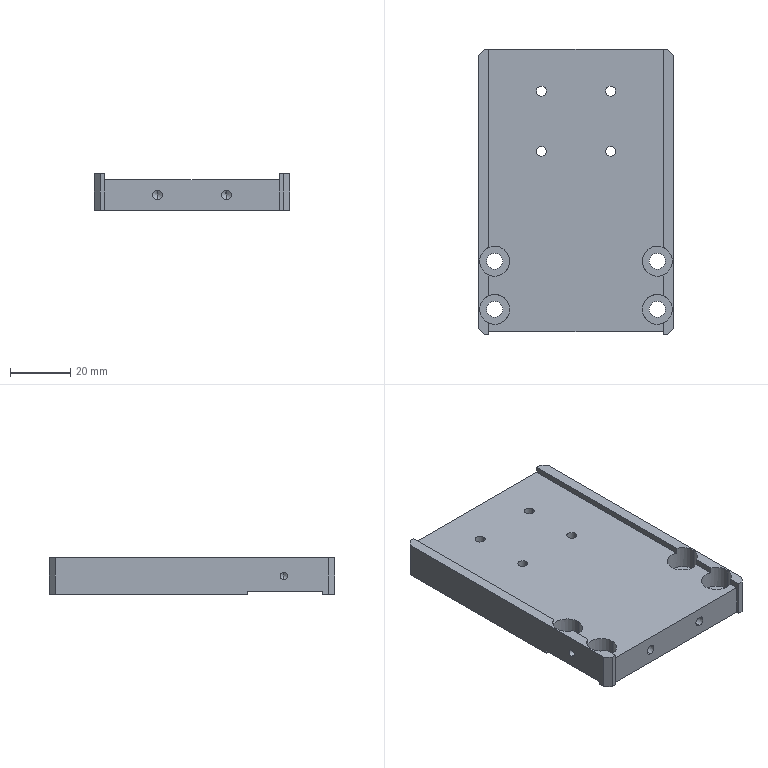Component | SolidWorks | 2018SOLIDWORKS1400000004-1 | 1 solid | 64 faces | box 65 x 95 x 12 mm | volume 57980 mm3 | cylinder 30 | plane 28 | cone 6 | commonest cylinder face diameters 3.3 x12 10 x8 5.3 x8 2.5 x2 | material 45 Steel
build123d program:
from build123d import *

# Parameters (mm, degrees)
SKETCH1_W                                            = 65
SKETCH1_H                                            = 95
BOSS_EXTRUDE1_DEPTH                                  = 12
SKETCH3_W                                            = 58
SKETCH3_H                                            = 95
CUT_EXTRUDE2_DEPTH                                   = 2
SKETCH4_W                                            = 58
SKETCH4_H                                            = 10
CUT_EXTRUDE3_DEPTH                                   = 1
SKETCH5_W                                            = 65
SKETCH5_H                                            = 25
CUT_EXTRUDE4_DEPTH                                   = 1
M4_TAPPED_HOLE1_D                                    = 3.3
M4_TAPPED_HOLE1_DEPTH                                = 10.1
M4_TAPPED_HOLE1_TIP                                  = 0.9914
M4_TAPPED_HOLE2_D                                    = 3.3
HOLE_SIZE_ACCORDING_TO_THE_TYPE_OF_HEX_S_D           = 5.3
HOLE_SIZE_ACCORDING_TO_THE_TYPE_OF_HEX_S_CBORE_D     = 10
HOLE_SIZE_ACCORDING_TO_THE_TYPE_OF_HEX_S_CBORE_DEPTH = 7.7
CHAMFER1_SIZE                                        = 2
M3_TAPPED_HOLE1_D                                    = 2.5
M3_TAPPED_HOLE1_DEPTH                                = 7.5
M3_TAPPED_HOLE1_TIP                                  = 0.7511


with BuildPart() as part:
    # Sketch1 → Boss-Extrude1 (new body)
    with BuildSketch(Plane.XY):
        Rectangle(SKETCH1_W, SKETCH1_H)
    extrude(amount=BOSS_EXTRUDE1_DEPTH)

    # Sketch3 → Cut-Extrude2 (cut)
    with BuildSketch(Plane.XY.offset(12)):
        Rectangle(SKETCH3_W, SKETCH3_H)
    extrude(amount=-CUT_EXTRUDE2_DEPTH, mode=Mode.SUBTRACT)

    # Sketch4 → Cut-Extrude3 (cut)
    with BuildSketch(Plane.XZ.offset(47.5)):
        with Locations((0, 5)):
            Rectangle(SKETCH4_W, SKETCH4_H)
    extrude(amount=-CUT_EXTRUDE3_DEPTH, mode=Mode.SUBTRACT)

    # Sketch5 → Cut-Extrude4 (cut)
    with BuildSketch(Plane(origin=(0, 0, 0), x_dir=(-1, 0, 0), z_dir=(0, 0, -1))):
        with Locations((0, -31)):
            Rectangle(SKETCH5_W, SKETCH5_H)
    extrude(amount=-CUT_EXTRUDE4_DEPTH, mode=Mode.SUBTRACT)

    # M4 Tapped Hole1
    with Locations(Plane(origin=(0, -46.5, 0), x_dir=(-1, 0, 0), z_dir=(0, -1, 0))):
        with Locations((-11.5, -5), (11.5, -5)):
            Hole(M4_TAPPED_HOLE1_D / 2, depth=M4_TAPPED_HOLE1_DEPTH)
            with Locations((0, 0, -(M4_TAPPED_HOLE1_DEPTH + M4_TAPPED_HOLE1_TIP / 2))):  # 118° drill point
                Cone(0, M4_TAPPED_HOLE1_D / 2, M4_TAPPED_HOLE1_TIP, mode=Mode.SUBTRACT)

    # M4 Tapped Hole2 (through all)
    with Locations(Plane.XY.offset(10)):
        with Locations((-11.5, 33.5), (11.5, 33.5), (-11.5, 13.5), (11.5, 13.5)):
            Hole(M4_TAPPED_HOLE2_D / 2)

    # Hole Size according to the type of hex s (through all)
    with Locations(Plane.XY.offset(12)):
        with Locations((27, -39), (27, -23), (-27, -23), (-27, -39)):
            CounterBoreHole(HOLE_SIZE_ACCORDING_TO_THE_TYPE_OF_HEX_S_D / 2, HOLE_SIZE_ACCORDING_TO_THE_TYPE_OF_HEX_S_CBORE_D / 2, HOLE_SIZE_ACCORDING_TO_THE_TYPE_OF_HEX_S_CBORE_DEPTH)

    # Chamfer1
    chamfer1_edges = [part.edges().sort_by_distance(p)[0] for p in [
        (32.5, -47.5, 6),
        (-32.5, -47.5, 6),
        (-32.5, 47.5, 6),
        (32.5, 47.5, 6),
    ]]
    chamfer(chamfer1_edges, length=CHAMFER1_SIZE)

    # M3 Tapped Hole1
    with Locations(Plane.ZY.offset(32.5)):
        with Locations((6, -30.5)):
            Hole(M3_TAPPED_HOLE1_D / 2, depth=M3_TAPPED_HOLE1_DEPTH)
            with Locations((0, 0, -(M3_TAPPED_HOLE1_DEPTH + M3_TAPPED_HOLE1_TIP / 2))):  # 118° drill point
                Cone(0, M3_TAPPED_HOLE1_D / 2, M3_TAPPED_HOLE1_TIP, mode=Mode.SUBTRACT)


solid = part.part

# Placed as in the assembly
solid = solid.moved(Location((163.212, -30, 174), (0, 0, 0)))